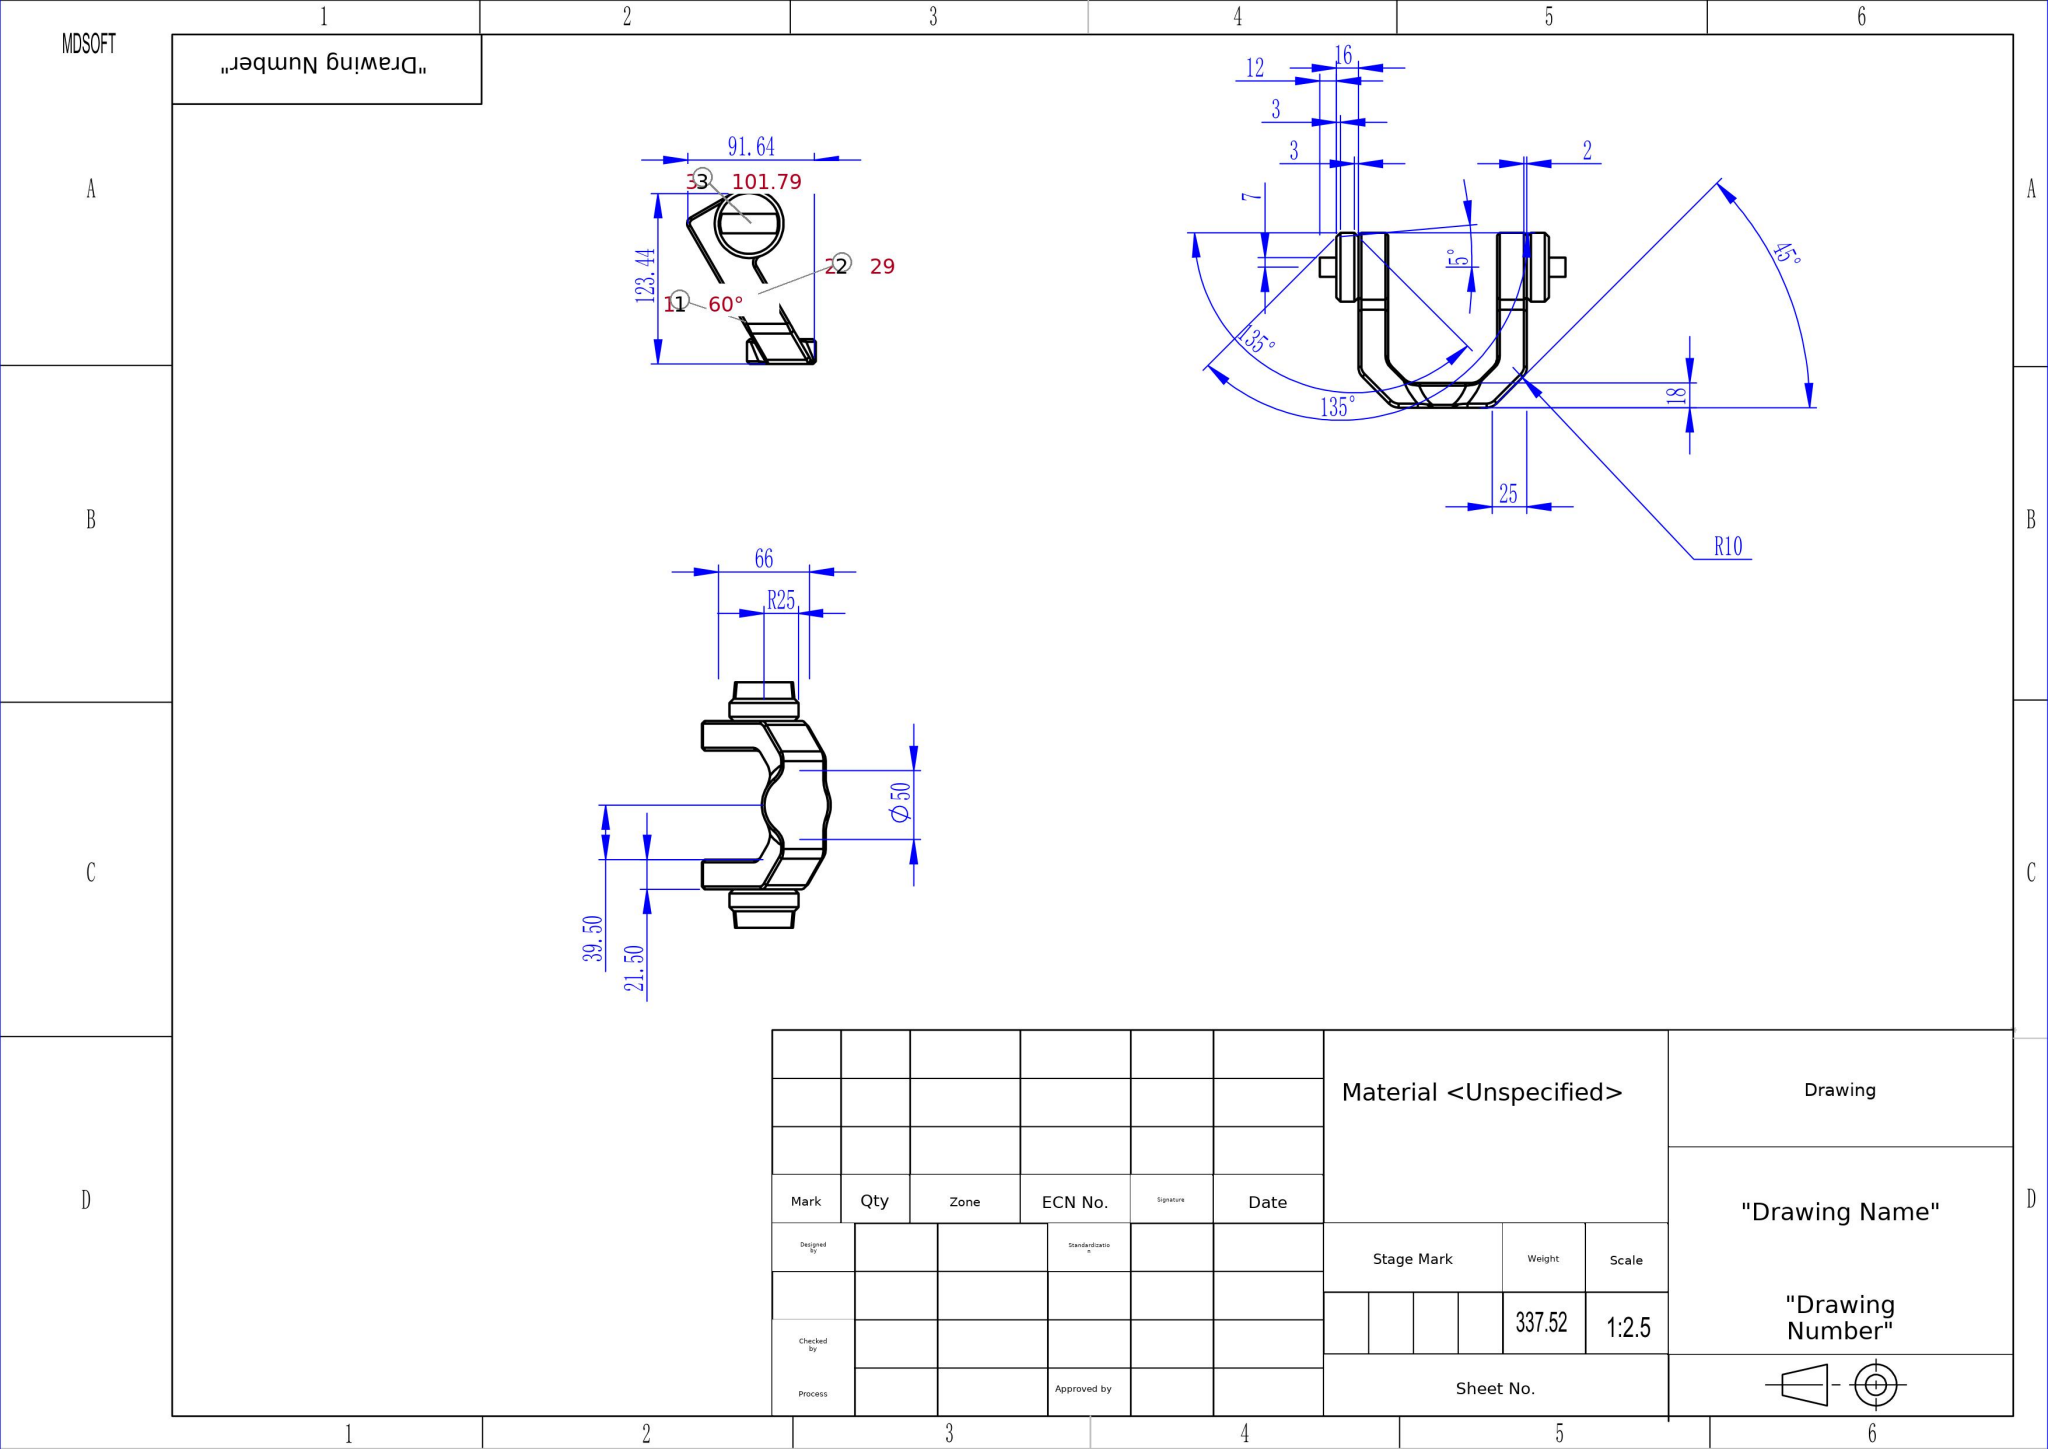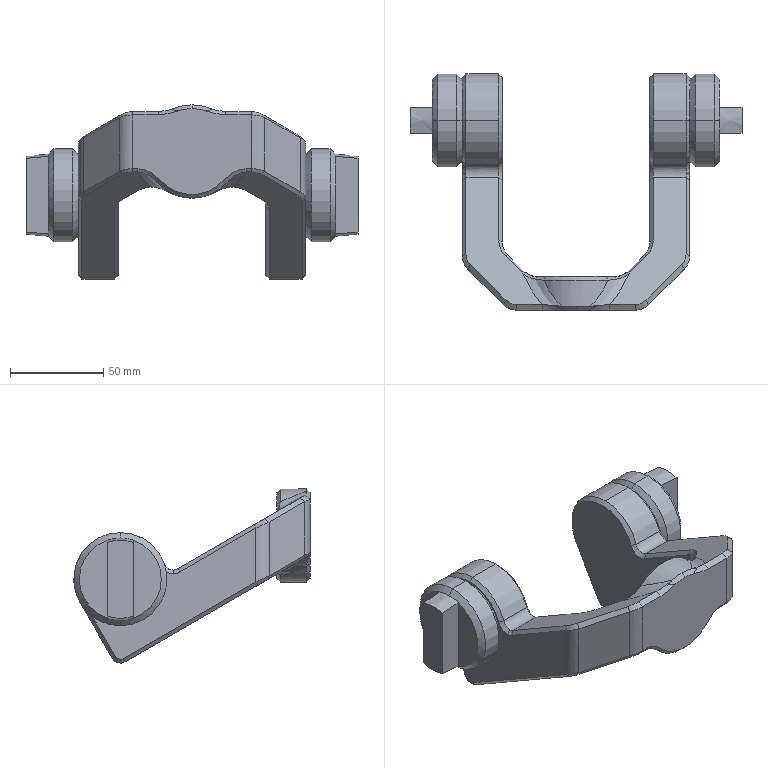Part | SolidWorks | mm | 1 solid | 147 faces | box 178 x 126.79 x 93.39 mm | volume 337536 mm3 | plane 50 | cone 38 | spline 32 | cylinder 27 | commonest cylinder face diameters 50 x15 20 x8 10 x4